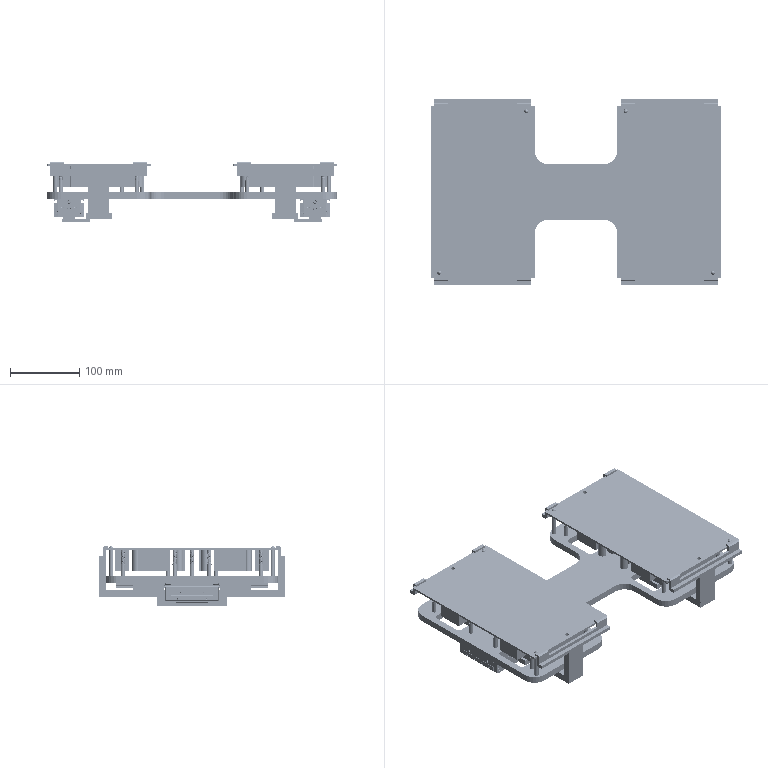Assembly | SolidWorks | mm | 49 component files | 49 solids | 4501 faces | box 420 x 270 x 87 mm | volume 2045000 mm3 | plane 2129 | cylinder 1222 | spline 802 | cone 340 | torus 8 | commonest cylinder face diameters 5 x396 6 x192 4.4 x44 3 x40 3.242 x40 3.5 x36 5.3 x36 6.5 x36
Bill of materials:
Gripper-2024-3-4-04 | 1 | AL6061 | Flat plate of uniform thickness with an H / dog-bone outline: two wide rounded-corner end regions joined by a narrower central web with filleted inside corners. Each end region has four rounded-rectangle through cutouts in a 2x2 arrangement (eight in total), and the plate has many small through holes near the perimeter and along the centre.
Gripper-2024-3-4-05 | 1 | AL6061 | L-section angle bar: a long horizontal leg with a short upright leg at one end. A shallow narrow groove or step line runs along the top of the long leg near its far edge.
Gripper-2024-3-4-06 | 1 | S45C | Flat block with an L-shaped (notched-rectangle) top outline and a stepped side profile: two plate sections offset in height, overlapping at a lap-type step.
Gripper-2024-3-4-07 | 1 | S45C | Long slender bar with a raised upright tab at each end. The tabs have chamfered or angled top edges, giving a Z-like or hooked end profile. There is a shallow relief on the underside at mid-length.
Gripper-2024-3-4-08 | 2 | S45C | Plain cylindrical pin or rod with a chamfered or domed tip at one end and a flat or slightly rounded opposite end.
HFD12X25(CL)_b | 1 |  | Compact rectangular block with a separate-looking top plate. The top face has a large circular recess and small holes. The end face has round ports, counterbored holes and hex-socket features, and U-shaped slots at two corners. Each long side has longitudinal grooves and small round holes.
HFD12X25(CL)_t | 2 |  | Rectangular block with a rectangular slot or channel running across its top, small shoulder steps along the upper sides, chamfered lower corners, and one round through hole in the vertical direction.
LinearGuideMGN12(HIWIN) | 1 | Chrome Stainless Steel | Long straight bar with a roughly rectangular cross-section that has large semicircular notches on both sides, small chamfers at the corners, and a small notch on top. A single row of evenly spaced holes runs along the centreline of the top face.
Mirror_HFD12X25(CL)_b | 1 |  | Rectangular block body with a separate-looking flat top plate. The top plate has rounded long edges and stepped ends. There are long grooves along the sides, U-shaped notches at the corners of the end face, and many small circular holes and recessed hex-socket features.
Mirror_HFD12X25(CL)_t | 1 |  | Small rectangular block. Its upper part is stepped: shoulders on both sides overhang a slightly narrower body, and a rectangular notch runs across the top. One round through hole passes vertically through the block.
Mirror_HFD12X25(CL)_t1 | 1 |  | Small rectangular block. Its upper part is stepped: shoulders on both sides overhang a slightly narrower body, and a rectangular notch runs across the top. One round through hole passes vertically through the block.
Mirror_Mirror_PNP110-M-H | 4 |  | Stepped cylindrical shaft. One end section carries a helical ridge or coil. Below it is a short larger-diameter collar, then a long plain cylindrical section, then a reduced neck with a groove, and a short end spigot.
Mirror_PNP110-M-H | 9 |  | Stepped cylindrical shaft. One end section carries a helical ridge or coil. Below it are a larger collar, a long plain section, a grooved neck, and a short end spigot.
MirroredGripper-2024-3-4-05 | 2 | AL6061 | L-section angle bar: a long horizontal leg with a short upright leg at one end. The top of the long leg has a shallow rectangular recessed step or pocket running along part of its length near the free end.
MirroredGripper-2024-3-4-06 | 2 | S45C | Flat block with an L-shaped (notched-rectangle) top outline and a stepped side profile: two plate sections offset in height, overlapping at a lap-type step.
MirroredGripper-2024-3-4-07 | 2 | S45C | Long slender prismatic bar with a stepped, roughly Z-shaped cross-section; the top has raised pads at both ends with a lower recessed span between them.
MirroredGripper-2024-3-4-08 | 2 | S45C | Plain solid cylindrical pin with a chamfered or rounded tapered tip at one end and a flat or slightly rounded opposite end.
MirroredLinearGuideMGN12(HIWIN) | 1 | Chrome Stainless Steel | Long straight rail-like bar with a row of evenly spaced holes through its top face and a longitudinal groove along each side.
MirroredMirroredGripper-2024-3-4-05 | 1 | AL6061 | L-shaped bracket: a long flat rectangular base with a rectangular upright wall at one end, plus a shallow step or rabbet along part of the base's top surface.
MirroredMirroredGripper-2024-3-4-06 | 1 | S45C | Stepped block made of two rectangular slabs: a larger, thicker slab and a smaller, thinner slab offset from it, giving an L-shaped plan and a stepped side profile.
MirroredMirroredGripper-2024-3-4-07 | 1 | S45C | Long slender prismatic bar with a stepped, roughly Z-shaped cross-section; the top has raised pads at both ends with a lower recessed span between them.
MirroredMirroredSliderMGN12H(HIWIN) | 1 | Gray Cast Iron | Rectangular block with a wide channel running lengthwise along its underside. Each channel wall has a semicircular groove with a cylindrical rod-like bead in it. The block has end sections, a small hole on the end face, and embossed or engraved text.
MirroredPCBBoard | 1 |  | Thin rectangular plate with four small through holes near the corners. Several rectangular blocks and some cylindrical features hang from its underside.
MirroredSliderMGN12H(HIWIN) | 2 | Gray Cast Iron | Rectangular block with a lengthwise channel on its underside, cylindrical beads in the channel-wall grooves, a longitudinal side groove, a small end-face hole, and embossed or engraved text on the end face.
PCBBoard | 1 |  | Thin rectangular plate with four small corner-area holes. Rectangular blocks and two short cylindrical posts project from its underside.
PNP110-M-H | 5 |  | Stepped cylindrical shaft with a helical wire-like coil around its upper section, a shoulder collar, a main shank, a necked groove, and a smaller-diameter end portion.
SliderMGN12H(HIWIN) | 1 | Gray Cast Iron | Rectangular block with a lengthwise channel on its underside, cylindrical beads in the channel-wall grooves, a longitudinal side groove, small holes and circular marks on the end face, and embossed or engraved text.
Mates:
1. width | PCBBoard-1 face at (-175.094, 118.231, 345) dir (0, 1, 0) | PCBBoard-1 face at (-175.094, -131.769, 345) dir (0, -1, 0) | Gripper-2024-3-4-04-1 face at (824.906, 118.231, 295) dir (0, 1, 0) | Gripper-2024-3-4-04-1 face at (824.906, -131.769, 295) dir (0, -1, 0)
2. coincident | Gripper-2024-3-4-04-1 face at (-175.094, -141.769, 305) dir (-1, 0, 0) | PCBBoard-1 face at (-175.094, 118.231, 345) dir (-1, 0, 0)
3. distance | PCBBoard-1 face at (-175.094, 118.231, 345) dir (0, 0, 1) | Gripper-2024-3-4-04-1 face at (-175.094, -141.769, 305) dir (0, 0, 1)
4. coincident | Gripper-2024-3-4-04-1 face at (-175.094, -141.769, 295) dir (0, 0, -1) | HFD12X25_CL-1/HFD12X25(CL)_b-1 face at (-164.351, 24.231, 295) dir (0, 0, 1)
5. width | HFD12X25_CL-1/HFD12X25(CL)_b-1 face at (-124.001, 32.231, 290.5) dir (0, 1, 0) | HFD12X25_CL-1/HFD12X25(CL)_b-1 face at (-124.001, -45.769, 290.5) dir (0, -1, 0) | Gripper-2024-3-4-04-1 face at (824.906, -131.769, 295) dir (0, -1, 0) | Gripper-2024-3-4-04-1 face at (824.906, 118.231, 295) dir (0, 1, 0)
6. coincident | Gripper-2024-3-4-04-1 face at (-175.094, -141.769, 295) dir (0, 0, -1) | LinearGuideMGN12(HIWIN)-1 face at (-98.294, -116.769, 295) dir (0, 0, 1)
7. distance | Gripper-2024-3-4-04-1 face at (824.906, -131.769, 295) dir (0, -1, 0) | LinearGuideMGN12(HIWIN)-1 face at (-106.094, -116.769, 289.5) dir (0, -1, 0)
8. coincident | LinearGuideMGN12(HIWIN)-1 face at (-94.394, -116.769, 287) dir (0, 0, -1) | SliderMGN12H(HIWIN)-1 face at (-94.094, -34.469, 287) dir (0, 0, 1)
9. concentric | LinearGuideMGN12(HIWIN)-1 face at (-106.094, -116.769, 289.5) dir (0, 1, 0) r 1.25 | SliderMGN12H(HIWIN)-1 face at (-106.094, -34.469, 289.5) dir (0, -1, 0) r 1.25
10. distance | Gripper-2024-3-4-05-1 face at (-115.094, -131.769, 330) dir (0, 1, 0) | Gripper-2024-3-4-04-1 face at (824.906, -131.769, 295) dir (0, -1, 0)
11. coincident | Gripper-2024-3-4-05-1 face at (-85.094, -141.769, 282) dir (0, 0, 1) | SliderMGN12H(HIWIN)-1 face at (-113.594, -46.769, 282) dir (0, 0, -1)
12. coincident | Gripper-2024-3-4-05-1 face at (-113.594, 79.231, 282) dir (1, 0, 0) | SliderMGN12H(HIWIN)-1 face at (-113.594, -46.769, 292) dir (-1, 0, 0)
13. distance | SliderMGN12H(HIWIN)-1 face at (-86.594, -46.769, 289) dir (0, 1, 0) | Gripper-2024-3-4-05-1 face at (-115.094, -6.769, 274) dir (0, 1, 0)
14. coincident | HFD12X25_CL-1/HFD12X25(CL)_t-2 face at (-134.901, -6.819, 266) dir (0, 0, -1) | Gripper-2024-3-4-06-1 face at (-153.651, -6.819, 266) dir (0, 0, 1)
15. coincident | HFD12X25_CL-1/HFD12X25(CL)_t-2 face at (-143.151, -6.819, 295) dir (0, 1, 0) | Gripper-2024-3-4-06-1 face at (-153.651, -6.819, 266) dir (0, 1, 0)
16. distance | HFD12X25_CL-1/HFD12X25(CL)_t-2 face at (-151.651, -6.819, 266.25) dir (-1, 0, 0) | Gripper-2024-3-4-06-1 face at (-153.651, -6.819, 266) dir (-1, 0, 0)
17. coincident | PCBBoard-1 face at (-175.094, -131.769, 345) dir (0, -1, 0) | Gripper-2024-3-4-07-1 face at (-30.094, -131.769, 328) dir (0, 1, 0)
18. coincident | PCBBoard-1 face at (-175.094, 118.231, 345) dir (0, 0, 1) | Gripper-2024-3-4-07-1 face at (-30.094, -128.769, 345) dir (0, 0, -1)
19. coincident | Gripper-2024-3-4-05-1 face at (-85.094, -141.769, 330) dir (1, 0, 0) | Gripper-2024-3-4-07-1 face at (-85.094, -141.769, 330) dir (-1, 0, 0)
20. concentric | Gripper-2024-3-4-04-1 face at (-163.094, -123.769, 303) dir (0, 0, 1) r 3 | Gripper-2024-3-4-08-1 face at (-163.094, -123.769, 348) dir (0, 0, -1) r 3
21. coincident | Gripper-2024-3-4-04-1 face at (-163.094, -123.769, 303) dir (0, 0, 1) | Gripper-2024-3-4-08-1 face at (-163.094, -123.769, 303) dir (0, 0, -1)
22. concentric | Gripper-2024-3-4-04-1 face at (-37.094, 110.231, 303) dir (0, 0, 1) r 3 | Gripper-2024-3-4-08-2 face at (-37.094, 110.231, 348) dir (0, 0, -1) r 3
23. coincident | Gripper-2024-3-4-04-1 face at (-37.094, 110.231, 303) dir (0, 0, 1) | Gripper-2024-3-4-08-2 face at (-37.094, 110.231, 303) dir (0, 0, -1)
24. distance | LinearGuideMGN12(HIWIN)-1 face at (-106.094, -116.769, 290.75) dir (-1, 0, 0) | Gripper-2024-3-4-04-1 face at (-175.094, -141.769, 305) dir (-1, 0, 0)
25. concentric | Gripper-2024-3-4-04-1 face at (-45.094, -106.769, 305) dir (0, 0, 1) r 2.5 | PNP110-M-H-1 face at (-45.094, -106.769, 444) dir (0, 0, 1) r 2.5
26. concentric | Gripper-2024-3-4-04-1 face at (-100.094, -6.769, 305) dir (0, 0, 1) r 2.5 | PNP110-M-H-5 face at (-100.094, -6.769, 444) dir (0, 0, 1) r 2.5
27. concentric | Gripper-2024-3-4-04-1 face at (-155.094, -31.769, 305) dir (0, 0, 1) r 2.5 | PNP110-M-H-3 face at (-155.094, -31.769, 444) dir (0, 0, 1) r 2.5
28. concentric | Gripper-2024-3-4-04-1 face at (-67.094, -41.769, 305) dir (0, 0, 1) r 2.5 | PNP110-M-H-4 face at (-67.094, -41.769, 444) dir (0, 0, 1) r 2.5
29. concentric | Gripper-2024-3-4-04-1 face at (-155.094, -106.769, 305) dir (0, 0, 1) r 2.5 | PNP110-M-H-2 face at (-155.094, -106.769, 444) dir (0, 0, 1) r 2.5
30. distance | PNP110-M-H-1 face at (-42.634, -104.645, 322) dir (0, 0, 1) | Gripper-2024-3-4-07-1 face at (-30.094, -128.769, 345) dir (0, 0, -1)
31. coincident | PNP110-M-H-1 face at (-42.634, -104.645, 322) dir (0, 0, 1) | PNP110-M-H-2 face at (-156.339, -103.767, 322) dir (0, 0, 1)
32. coincident | PNP110-M-H-2 face at (-156.339, -103.767, 322) dir (0, 0, 1) | PNP110-M-H-3 face at (-156.339, -28.767, 322) dir (0, 0, 1)
33. coincident | PNP110-M-H-1 face at (-42.634, -104.645, 322) dir (0, 0, 1) | PNP110-M-H-5 face at (-101.339, -3.767, 322) dir (0, 0, 1)
34. coincident | PNP110-M-H-1 face at (-42.634, -104.645, 322) dir (0, 0, 1) | PNP110-M-H-4 face at (-68.339, -38.767, 322) dir (0, 0, 1)